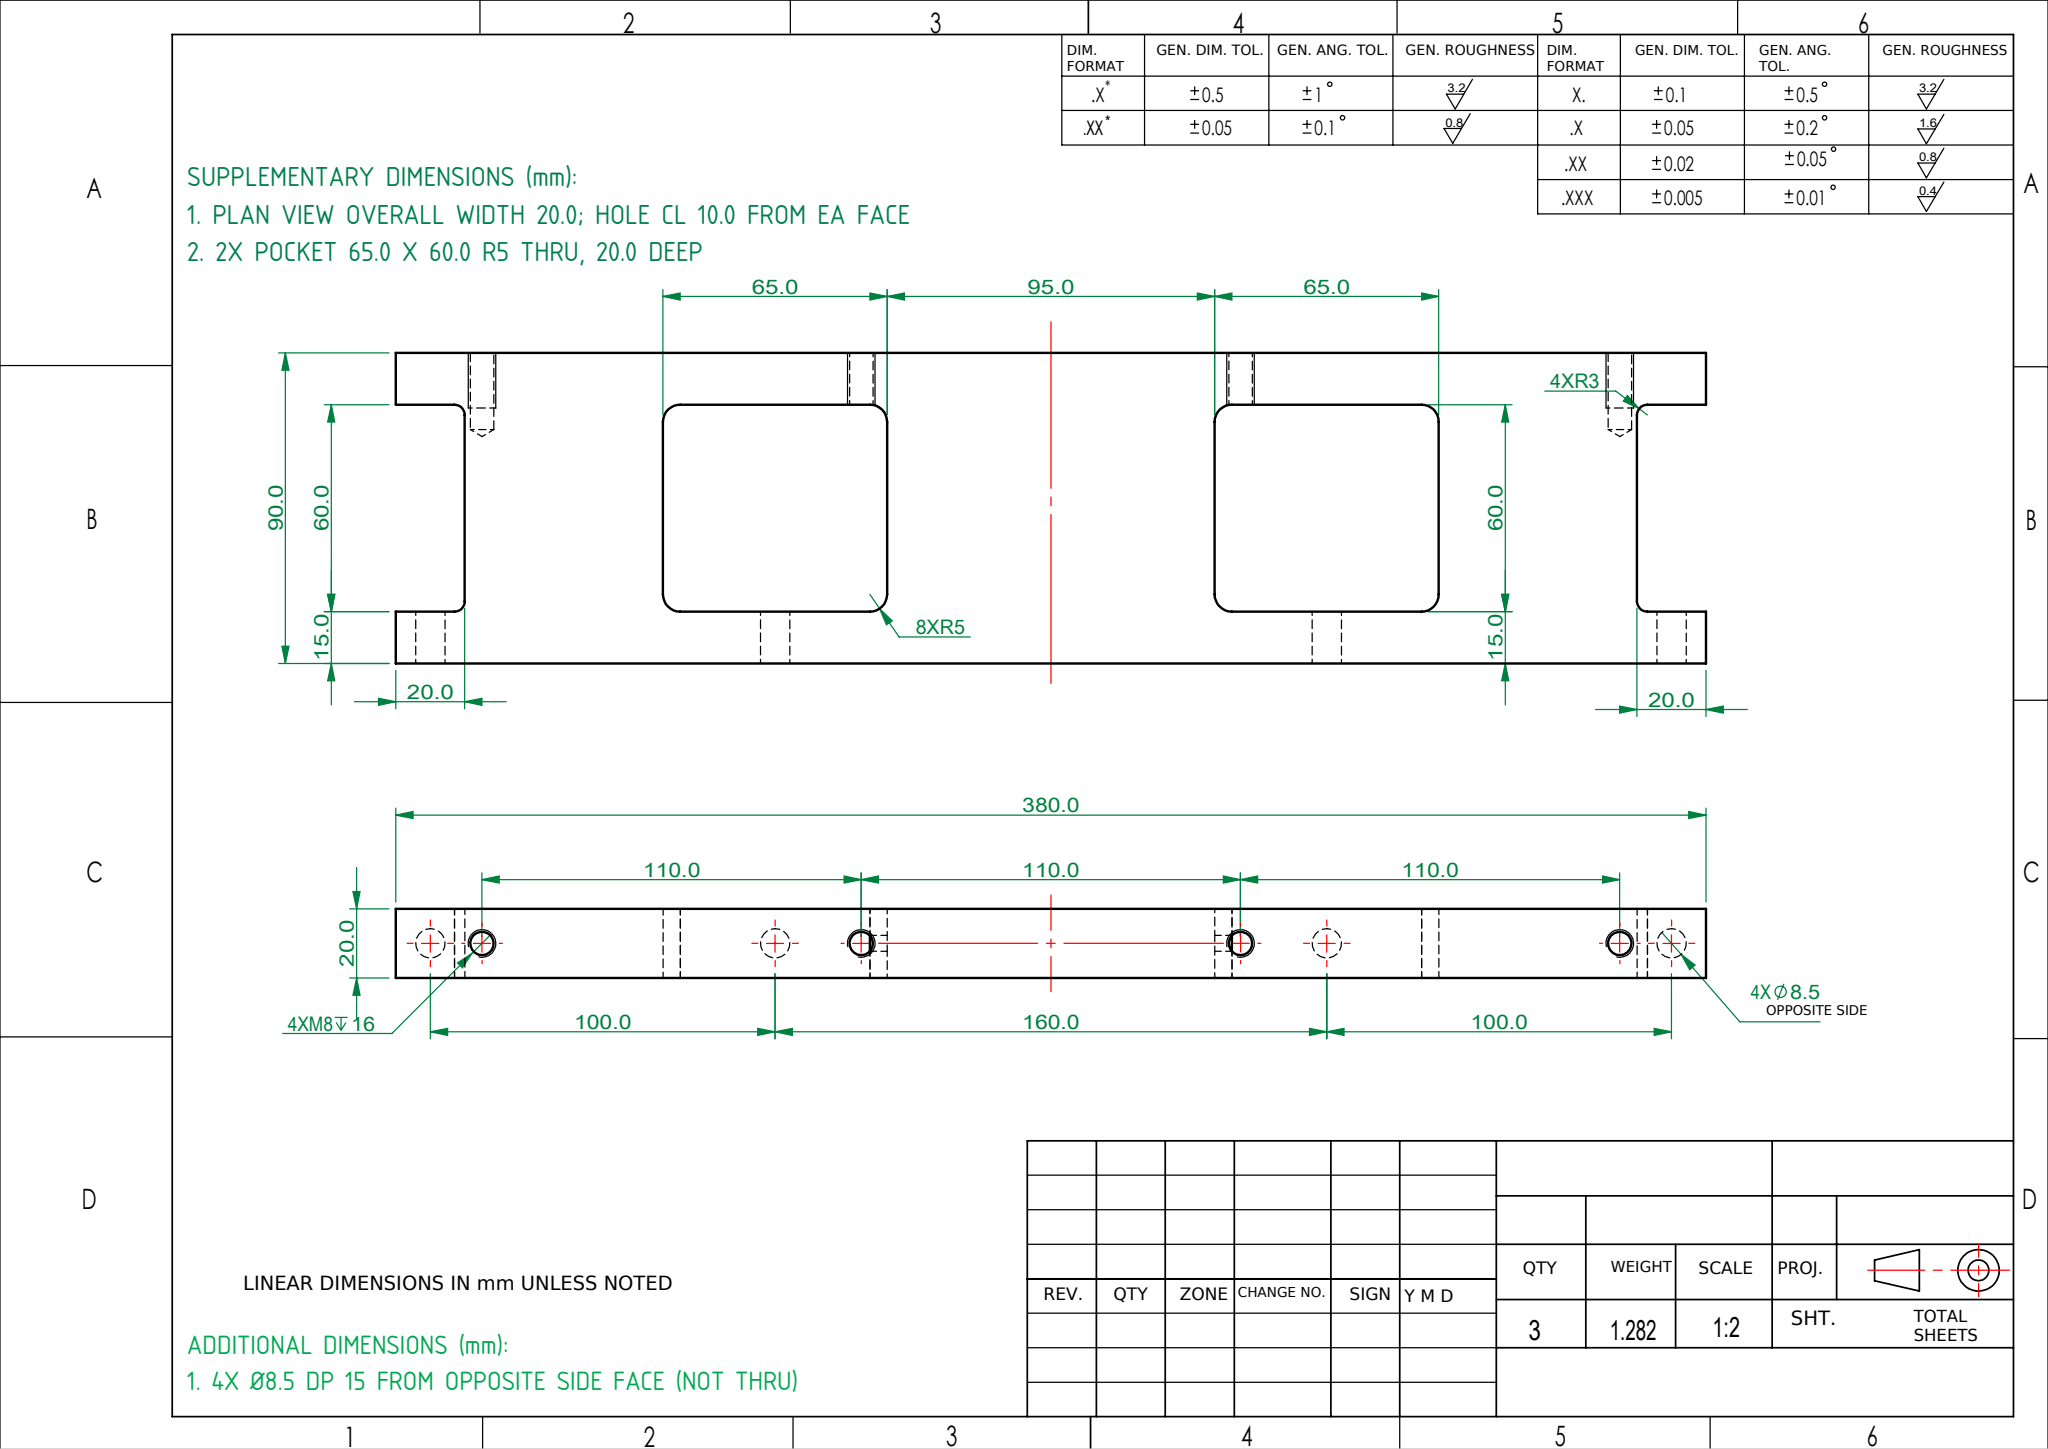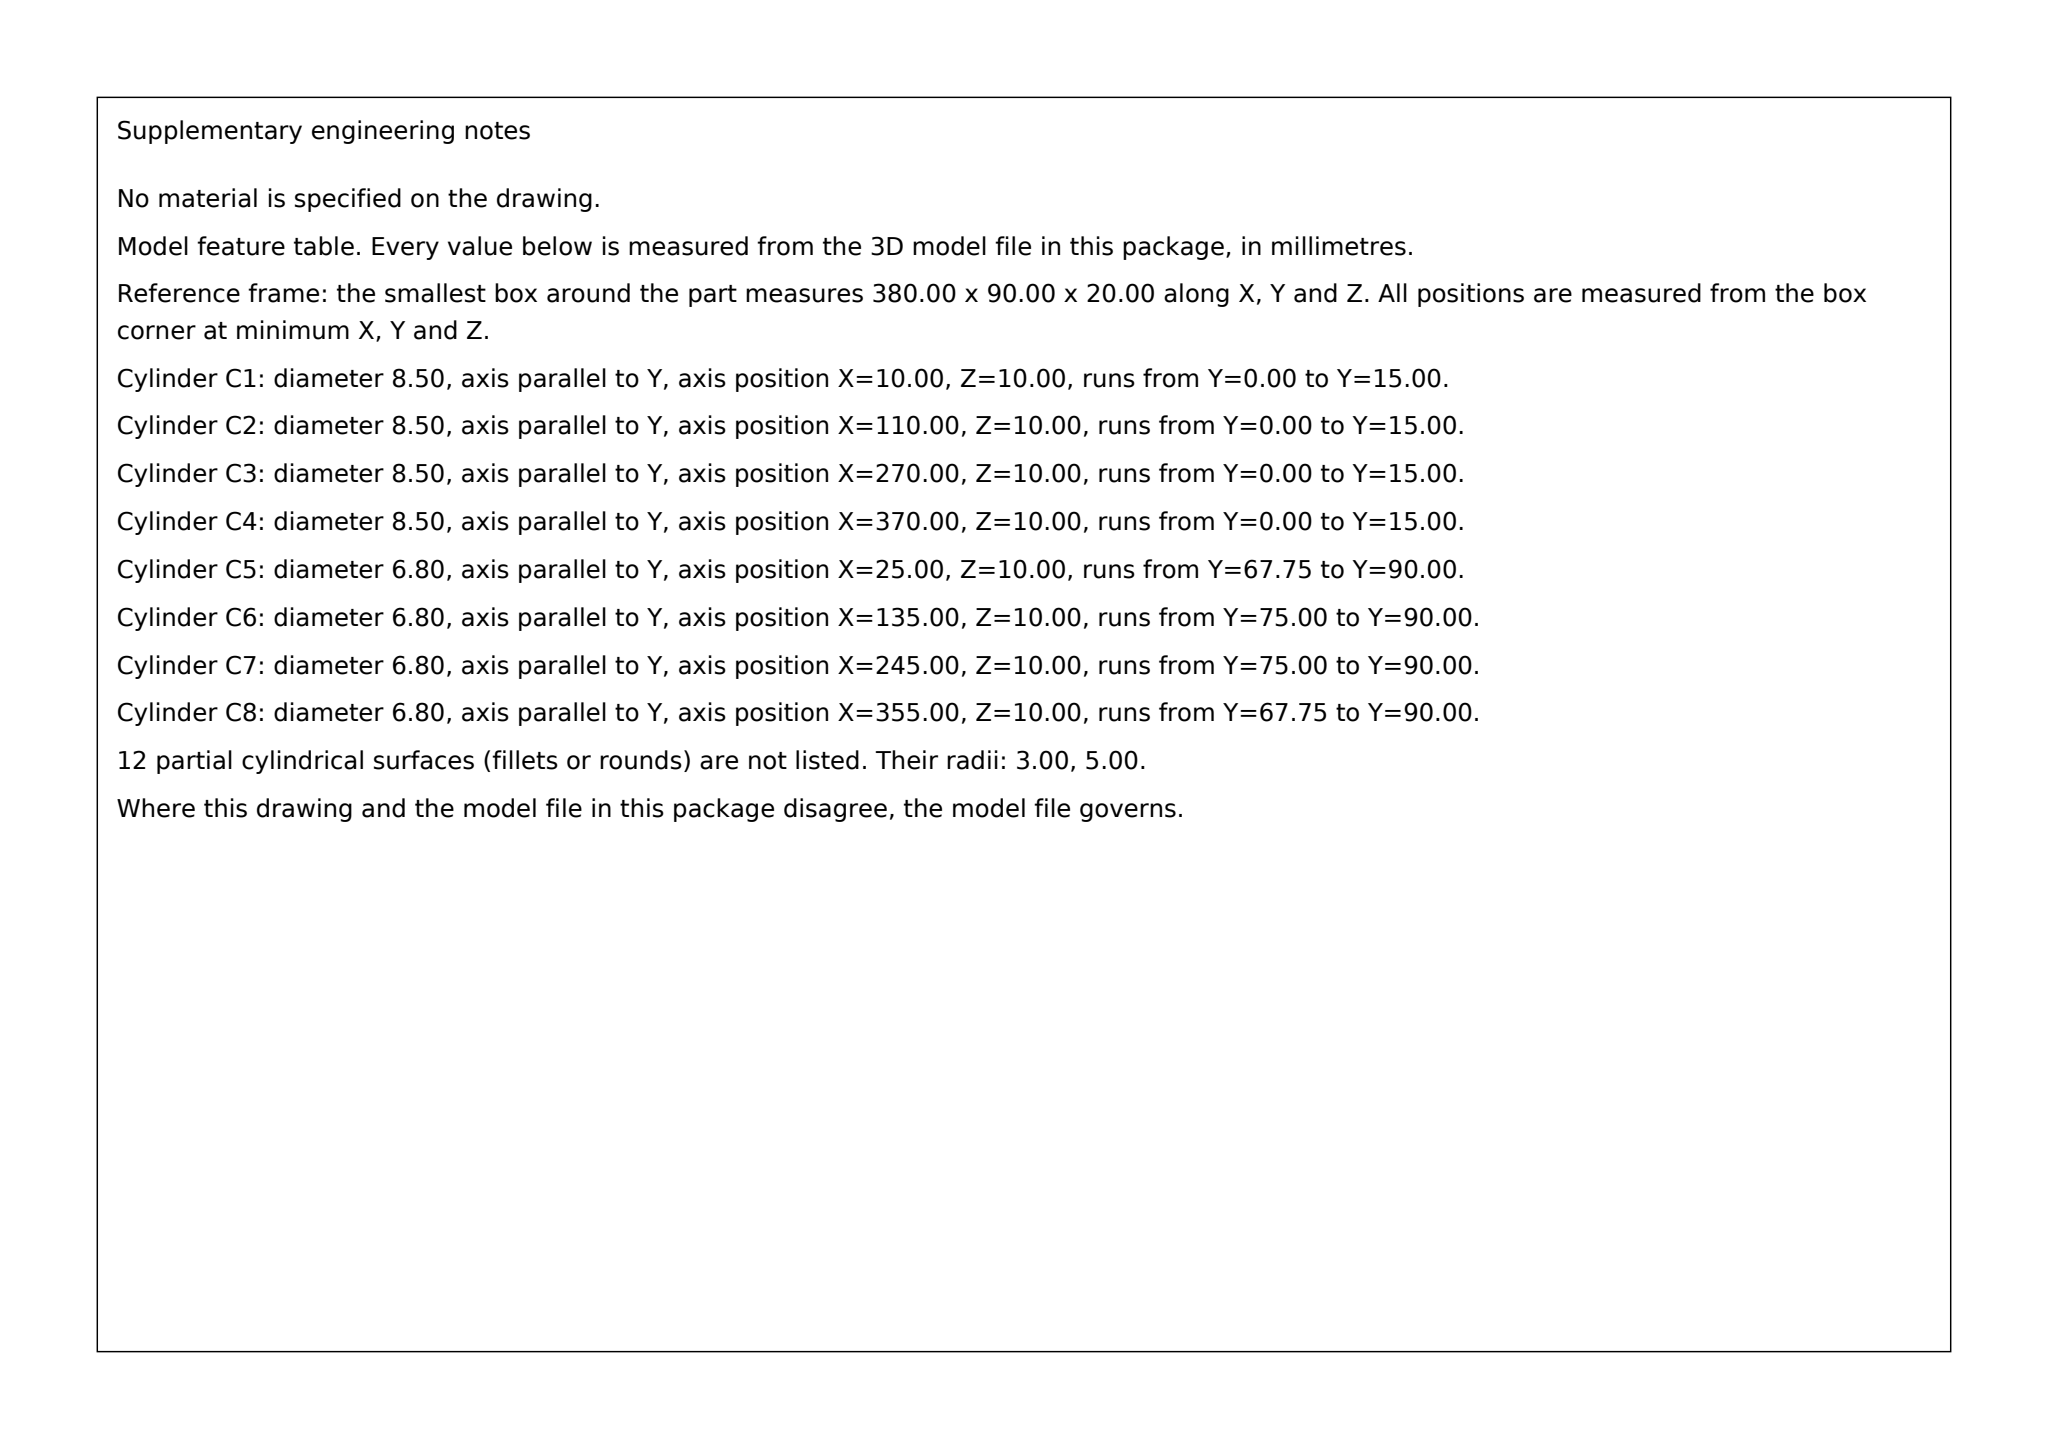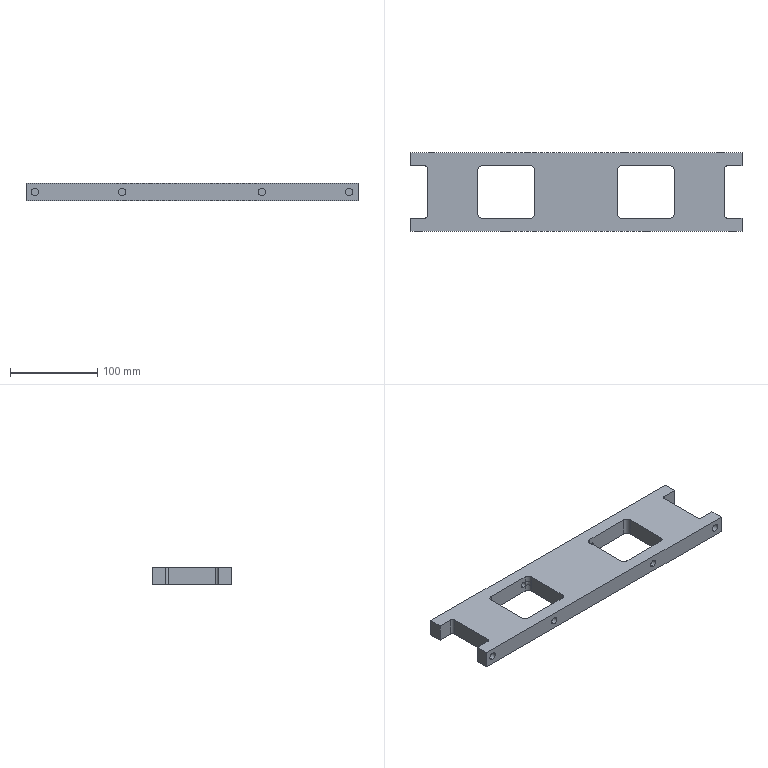Part | SolidWorks | mm | 1 solid | 58 faces | box 380 x 90 x 20 mm | volume 474851 mm3 | cylinder 30 | plane 22 | cone 4 | spline 2 | commonest cylinder face diameters 10 x10 8.5 x8 6.8 x8 6 x4